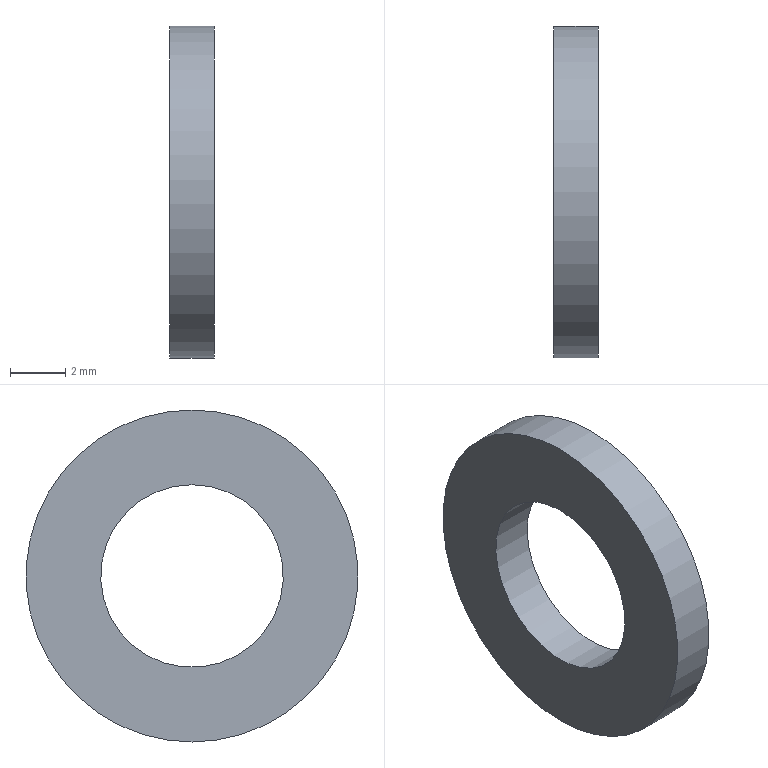Component | NX | GB-T95-2002_M6 | 1 solid | 4 faces | box 1.6 x 12 x 12 mm | volume 126 mm3 | cylinder 2 | plane 2 | commonest cylinder face diameters 12 x1 6.6 x1
STEP:
#1=CARTESIAN_POINT('',(0.,0.,0.));
#2=DIRECTION('',(0.,0.,1.));
#3=DIRECTION('',(1.,0.,0.));
#4=AXIS2_PLACEMENT_3D('',#1,#2,#3);
#5=CARTESIAN_POINT('',(58.6,-43.25,-10.5));
#6=VERTEX_POINT('',#5);
#7=CARTESIAN_POINT('',(58.6,-43.25,-16.5));
#8=DIRECTION('',(-1.,0.,0.));
#9=DIRECTION('',(0.,0.,1.));
#10=AXIS2_PLACEMENT_3D('',#7,#8,#9);
#11=CIRCLE('',#10,6.);
#12=CARTESIAN_POINT('',(57.,-43.25,-16.5));
#13=DIRECTION('',(-1.,0.,0.));
#14=DIRECTION('',(0.,0.,1.));
#15=AXIS2_PLACEMENT_3D('',#12,#13,#14);
#16=CYLINDRICAL_SURFACE('',#15,6.);
#17=CARTESIAN_POINT('',(0.,-1.6));
#18=DIRECTION('',(1.,0.));
#19=VECTOR('',#18,1.);
#20=LINE('',#17,#19);
#21=(GEOMETRIC_REPRESENTATION_CONTEXT(2)PARAMETRIC_REPRESENTATION_CONTEXT()REPRESENTATION_CONTEXT('',''));
#22=DEFINITIONAL_REPRESENTATION('',(#20),#21);
#23=PCURVE('',#16,#22);
#24=CARTESIAN_POINT('',(58.6,-43.25,-22.5));
#25=DIRECTION('',(1.,0.,0.));
#26=DIRECTION('',(0.,0.,-1.));
#27=AXIS2_PLACEMENT_3D('',#24,#25,#26);
#28=PLANE('',#27);
#29=CARTESIAN_POINT('',(-12.,0.));
#30=CARTESIAN_POINT('',(-12.,10.392));
#31=CARTESIAN_POINT('',(-3.,5.196));
#32=CARTESIAN_POINT('',(6.,0.));
#33=CARTESIAN_POINT('',(-3.,-5.196));
#34=CARTESIAN_POINT('',(-12.,-10.392));
#35=CARTESIAN_POINT('',(-12.,0.));
#36=(BOUNDED_CURVE()B_SPLINE_CURVE(2,(#29,#30,#31,#32,#33,#34,#35),.UNSPECIFIED.,.T.,.F.)B_SPLINE_CURVE_WITH_KNOTS((1,2,2,2,2,1),(-2.094,0.,2.094,4.189,6.283,8.378),.UNSPECIFIED.)CURVE()GEOMETRIC_REPRESENTATION_ITEM()RATIONAL_B_SPLINE_CURVE((1.,0.5,1.,0.5,1.,0.5,1.))REPRESENTATION_ITEM(''));
#37=(GEOMETRIC_REPRESENTATION_CONTEXT(2)PARAMETRIC_REPRESENTATION_CONTEXT()REPRESENTATION_CONTEXT('',''));
#38=DEFINITIONAL_REPRESENTATION('',(#36),#37);
#39=PCURVE('',#28,#38);
#40=SURFACE_CURVE('',#11,(#23,#39),.PCURVE_S1.);
#41=EDGE_CURVE('',#6,#6,#40,.T.);
#42=ORIENTED_EDGE('',*,*,#41,.T.);
#43=CARTESIAN_POINT('',(57.,-43.25,-10.5));
#44=VERTEX_POINT('',#43);
#45=CARTESIAN_POINT('',(58.6,-43.25,-10.5));
#46=CARTESIAN_POINT('',(57.,-43.25,-10.5));
#47=B_SPLINE_CURVE_WITH_KNOTS('',1,(#45,#46),.UNSPECIFIED.,.F.,.F.,(2,2),(-1.6,0.),.PIECEWISE_BEZIER_KNOTS.);
#48=CARTESIAN_POINT('',(6.283,0.));
#49=DIRECTION('',(0.,1.));
#50=VECTOR('',#49,1.);
#51=LINE('',#48,#50);
#52=(GEOMETRIC_REPRESENTATION_CONTEXT(2)PARAMETRIC_REPRESENTATION_CONTEXT()REPRESENTATION_CONTEXT('',''));
#53=DEFINITIONAL_REPRESENTATION('',(#51),#52);
#54=PCURVE('',#16,#53);
#55=CARTESIAN_POINT('',(0.,0.));
#56=DIRECTION('',(0.,1.));
#57=VECTOR('',#56,1.);
#58=LINE('',#55,#57);
#59=(GEOMETRIC_REPRESENTATION_CONTEXT(2)PARAMETRIC_REPRESENTATION_CONTEXT()REPRESENTATION_CONTEXT('',''));
#60=DEFINITIONAL_REPRESENTATION('',(#58),#59);
#61=PCURVE('',#16,#60);
#62=SEAM_CURVE('',#47,(#54,#61),.PCURVE_S1.);
#63=EDGE_CURVE('',#6,#44,#62,.T.);
#64=ORIENTED_EDGE('',*,*,#63,.T.);
#65=CARTESIAN_POINT('',(57.,-43.25,-16.5));
#66=DIRECTION('',(-1.,0.,0.));
#67=DIRECTION('',(0.,0.,1.));
#68=AXIS2_PLACEMENT_3D('',#65,#66,#67);
#69=CIRCLE('',#68,6.);
#70=CARTESIAN_POINT('',(0.,0.));
#71=DIRECTION('',(1.,0.));
#72=VECTOR('',#71,1.);
#73=LINE('',#70,#72);
#74=(GEOMETRIC_REPRESENTATION_CONTEXT(2)PARAMETRIC_REPRESENTATION_CONTEXT()REPRESENTATION_CONTEXT('',''));
#75=DEFINITIONAL_REPRESENTATION('',(#73),#74);
#76=PCURVE('',#16,#75);
#77=CARTESIAN_POINT('',(57.,-43.25,-19.8));
#78=DIRECTION('',(-1.,0.,0.));
#79=DIRECTION('',(0.,0.,1.));
#80=AXIS2_PLACEMENT_3D('',#77,#78,#79);
#81=PLANE('',#80);
#82=CARTESIAN_POINT('',(3.3,0.));
#83=DIRECTION('',(1.,0.));
#84=AXIS2_PLACEMENT_2D('',#82,#83);
#85=CIRCLE('',#84,6.);
#86=(GEOMETRIC_REPRESENTATION_CONTEXT(2)PARAMETRIC_REPRESENTATION_CONTEXT()REPRESENTATION_CONTEXT('',''));
#87=DEFINITIONAL_REPRESENTATION('',(#85),#86);
#88=PCURVE('',#81,#87);
#89=SURFACE_CURVE('',#69,(#76,#88),.PCURVE_S1.);
#90=EDGE_CURVE('',#44,#44,#89,.T.);
#91=ORIENTED_EDGE('',*,*,#90,.F.);
#92=ORIENTED_EDGE('',*,*,#63,.F.);
#93=EDGE_LOOP('',(#42,#64,#91,#92));
#94=FACE_BOUND('',#93,.T.);
#95=ADVANCED_FACE('',(#94),#16,.T.);
#96=CARTESIAN_POINT('',(58.6,-43.25,-13.2));
#97=VERTEX_POINT('',#96);
#98=CARTESIAN_POINT('',(58.6,-43.25,-16.5));
#99=DIRECTION('',(-1.,0.,0.));
#100=DIRECTION('',(0.,0.,1.));
#101=AXIS2_PLACEMENT_3D('',#98,#99,#100);
#102=CIRCLE('',#101,3.3);
#103=CARTESIAN_POINT('',(-9.3,0.));
#104=CARTESIAN_POINT('',(-9.3,5.716));
#105=CARTESIAN_POINT('',(-4.35,2.858));
#106=CARTESIAN_POINT('',(0.6,0.));
#107=CARTESIAN_POINT('',(-4.35,-2.858));
#108=CARTESIAN_POINT('',(-9.3,-5.716));
#109=CARTESIAN_POINT('',(-9.3,0.));
#110=(BOUNDED_CURVE()B_SPLINE_CURVE(2,(#103,#104,#105,#106,#107,#108,#109),.UNSPECIFIED.,.T.,.F.)B_SPLINE_CURVE_WITH_KNOTS((1,2,2,2,2,1),(-2.094,0.,2.094,4.189,6.283,8.378),.UNSPECIFIED.)CURVE()GEOMETRIC_REPRESENTATION_ITEM()RATIONAL_B_SPLINE_CURVE((1.,0.5,1.,0.5,1.,0.5,1.))REPRESENTATION_ITEM(''));
#111=(GEOMETRIC_REPRESENTATION_CONTEXT(2)PARAMETRIC_REPRESENTATION_CONTEXT()REPRESENTATION_CONTEXT('',''));
#112=DEFINITIONAL_REPRESENTATION('',(#110),#111);
#113=PCURVE('',#28,#112);
#114=CARTESIAN_POINT('',(57.,-43.25,-16.5));
#115=DIRECTION('',(-1.,0.,0.));
#116=DIRECTION('',(0.,0.,1.));
#117=AXIS2_PLACEMENT_3D('',#114,#115,#116);
#118=CYLINDRICAL_SURFACE('',#117,3.3);
#119=CARTESIAN_POINT('',(0.,-1.6));
#120=DIRECTION('',(1.,0.));
#121=VECTOR('',#120,1.);
#122=LINE('',#119,#121);
#123=(GEOMETRIC_REPRESENTATION_CONTEXT(2)PARAMETRIC_REPRESENTATION_CONTEXT()REPRESENTATION_CONTEXT('',''));
#124=DEFINITIONAL_REPRESENTATION('',(#122),#123);
#125=PCURVE('',#118,#124);
#126=SURFACE_CURVE('',#102,(#113,#125),.PCURVE_S1.);
#127=EDGE_CURVE('',#97,#97,#126,.T.);
#128=ORIENTED_EDGE('',*,*,#127,.T.);
#129=EDGE_LOOP('',(#128));
#130=FACE_BOUND('',#129,.T.);
#131=ORIENTED_EDGE('',*,*,#41,.F.);
#132=EDGE_LOOP('',(#131));
#133=FACE_BOUND('',#132,.T.);
#134=ADVANCED_FACE('',(#130,#133),#28,.T.);
#135=CARTESIAN_POINT('',(57.,-43.25,-13.2));
#136=VERTEX_POINT('',#135);
#137=CARTESIAN_POINT('',(57.,-43.25,-16.5));
#138=DIRECTION('',(-1.,0.,0.));
#139=DIRECTION('',(0.,0.,1.));
#140=AXIS2_PLACEMENT_3D('',#137,#138,#139);
#141=CIRCLE('',#140,3.3);
#142=CARTESIAN_POINT('',(0.,0.));
#143=DIRECTION('',(1.,0.));
#144=VECTOR('',#143,1.);
#145=LINE('',#142,#144);
#146=(GEOMETRIC_REPRESENTATION_CONTEXT(2)PARAMETRIC_REPRESENTATION_CONTEXT()REPRESENTATION_CONTEXT('',''));
#147=DEFINITIONAL_REPRESENTATION('',(#145),#146);
#148=PCURVE('',#118,#147);
#149=CARTESIAN_POINT('',(3.3,0.));
#150=DIRECTION('',(1.,0.));
#151=AXIS2_PLACEMENT_2D('',#149,#150);
#152=CIRCLE('',#151,3.3);
#153=(GEOMETRIC_REPRESENTATION_CONTEXT(2)PARAMETRIC_REPRESENTATION_CONTEXT()REPRESENTATION_CONTEXT('',''));
#154=DEFINITIONAL_REPRESENTATION('',(#152),#153);
#155=PCURVE('',#81,#154);
#156=SURFACE_CURVE('',#141,(#148,#155),.PCURVE_S1.);
#157=EDGE_CURVE('',#136,#136,#156,.T.);
#158=ORIENTED_EDGE('',*,*,#157,.F.);
#159=CARTESIAN_POINT('',(58.6,-43.25,-13.2));
#160=CARTESIAN_POINT('',(57.,-43.25,-13.2));
#161=B_SPLINE_CURVE_WITH_KNOTS('',1,(#159,#160),.UNSPECIFIED.,.F.,.F.,(2,2),(-1.6,0.),.PIECEWISE_BEZIER_KNOTS.);
#162=CARTESIAN_POINT('',(0.,0.));
#163=DIRECTION('',(0.,1.));
#164=VECTOR('',#163,1.);
#165=LINE('',#162,#164);
#166=(GEOMETRIC_REPRESENTATION_CONTEXT(2)PARAMETRIC_REPRESENTATION_CONTEXT()REPRESENTATION_CONTEXT('',''));
#167=DEFINITIONAL_REPRESENTATION('',(#165),#166);
#168=PCURVE('',#118,#167);
#169=CARTESIAN_POINT('',(6.283,0.));
#170=DIRECTION('',(0.,1.));
#171=VECTOR('',#170,1.);
#172=LINE('',#169,#171);
#173=(GEOMETRIC_REPRESENTATION_CONTEXT(2)PARAMETRIC_REPRESENTATION_CONTEXT()REPRESENTATION_CONTEXT('',''));
#174=DEFINITIONAL_REPRESENTATION('',(#172),#173);
#175=PCURVE('',#118,#174);
#176=SEAM_CURVE('',#161,(#168,#175),.PCURVE_S1.);
#177=EDGE_CURVE('',#97,#136,#176,.T.);
#178=ORIENTED_EDGE('',*,*,#177,.F.);
#179=ORIENTED_EDGE('',*,*,#127,.T.);
#180=ORIENTED_EDGE('',*,*,#177,.T.);
#181=EDGE_LOOP('',(#158,#178,#179,#180));
#182=FACE_BOUND('',#181,.F.);
#183=ADVANCED_FACE('',(#182),#118,.F.);
#184=ORIENTED_EDGE('',*,*,#90,.T.);
#185=EDGE_LOOP('',(#184));
#186=FACE_BOUND('',#185,.T.);
#187=ORIENTED_EDGE('',*,*,#157,.F.);
#188=EDGE_LOOP('',(#187));
#189=FACE_BOUND('',#188,.T.);
#190=ADVANCED_FACE('',(#186,#189),#81,.T.);
#191=CLOSED_SHELL('',(#95,#134,#183,#190));
#192=MANIFOLD_SOLID_BREP('',#191);
#193=(LENGTH_UNIT()NAMED_UNIT(*)SI_UNIT(.MILLI.,.METRE.));
#194=UNCERTAINTY_MEASURE_WITH_UNIT(LENGTH_MEASURE(0.00001),#193,'','');
#195=(NAMED_UNIT(*)PLANE_ANGLE_UNIT()SI_UNIT($,.RADIAN.));
#196=(NAMED_UNIT(*)SI_UNIT($,.STERADIAN.)SOLID_ANGLE_UNIT());
#197=(GEOMETRIC_REPRESENTATION_CONTEXT(3)GLOBAL_UNCERTAINTY_ASSIGNED_CONTEXT((#194))GLOBAL_UNIT_ASSIGNED_CONTEXT((#193,#195,#196))REPRESENTATION_CONTEXT('',''));
#198=ADVANCED_BREP_SHAPE_REPRESENTATION('',(#4,#192),#197);